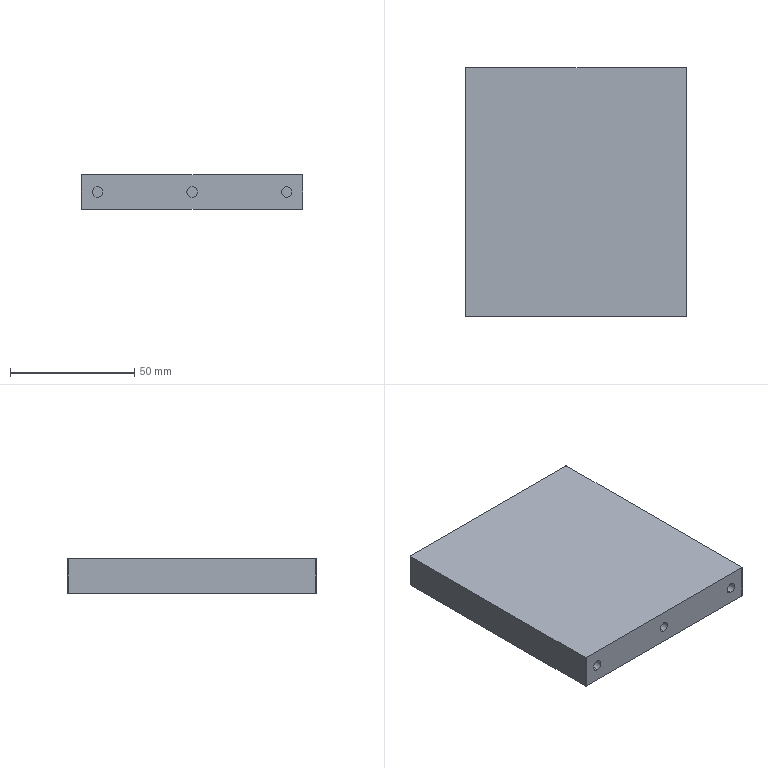CAM job | Mastercam | mm | 8 operations | part box 89 x 100 x 14
1. Facing | 20 - 63 平铣刀
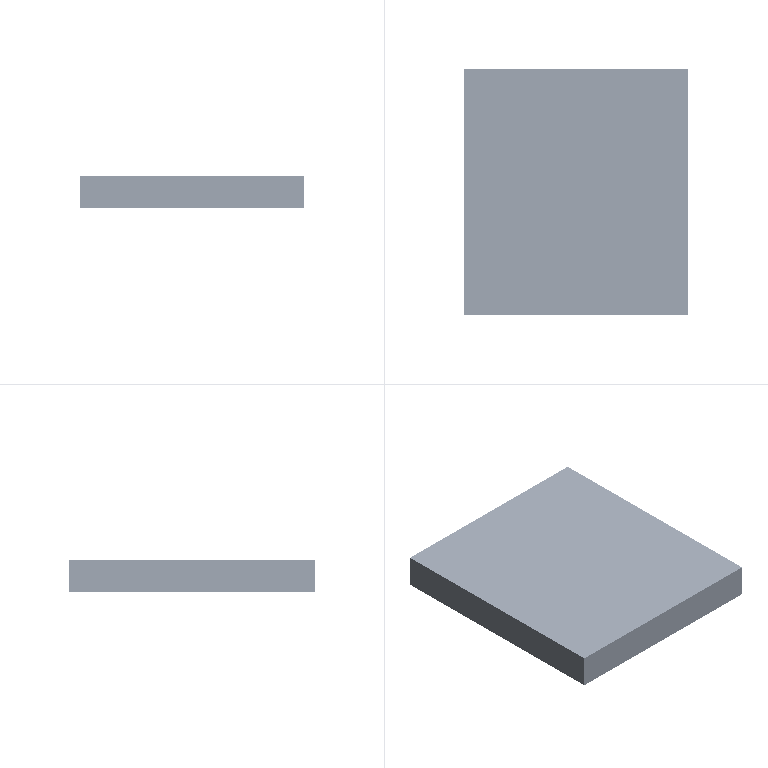2. Contour (Ramp) | 12 - 12 平铣刀
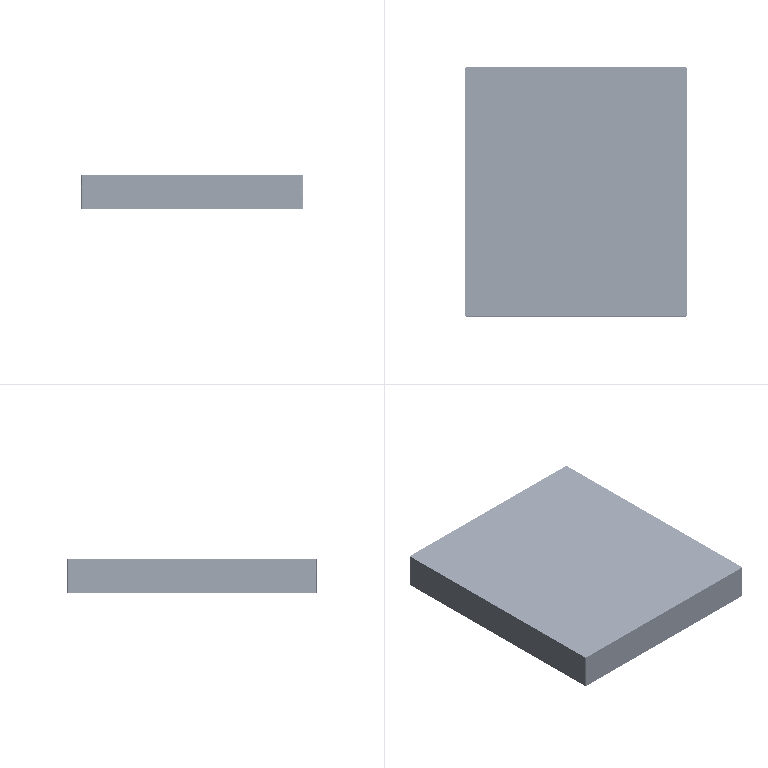3. Contour (2D) | 12 - 12 平铣刀
4. Contour (2D chamfer) | 7 - 4 倒角刀
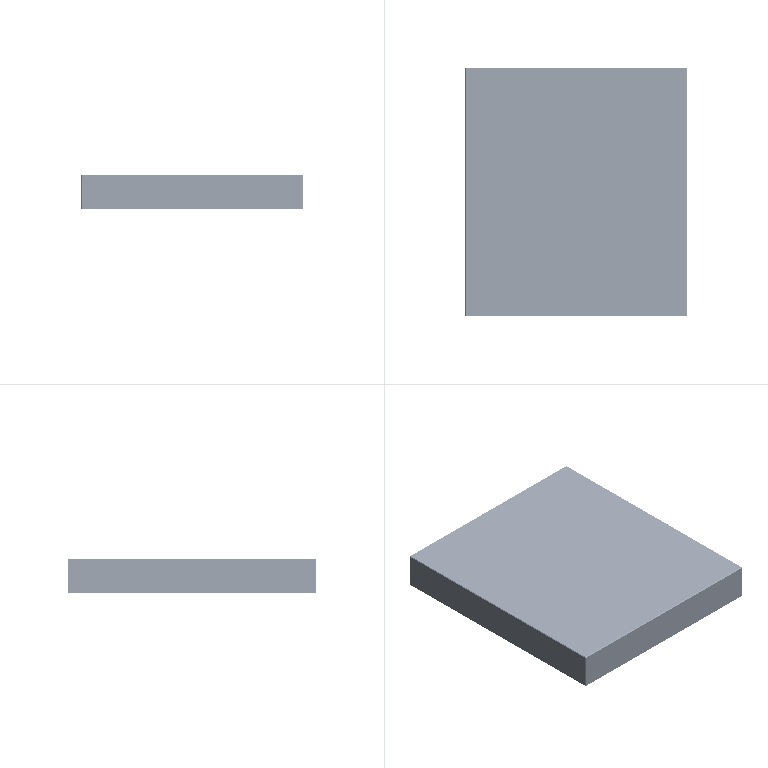5. Facing | 20 - 63 平铣刀
6. Contour (2D chamfer) | 7 - 4 倒角刀
7. Drill/Counterbore | 7 - 4 倒角刀
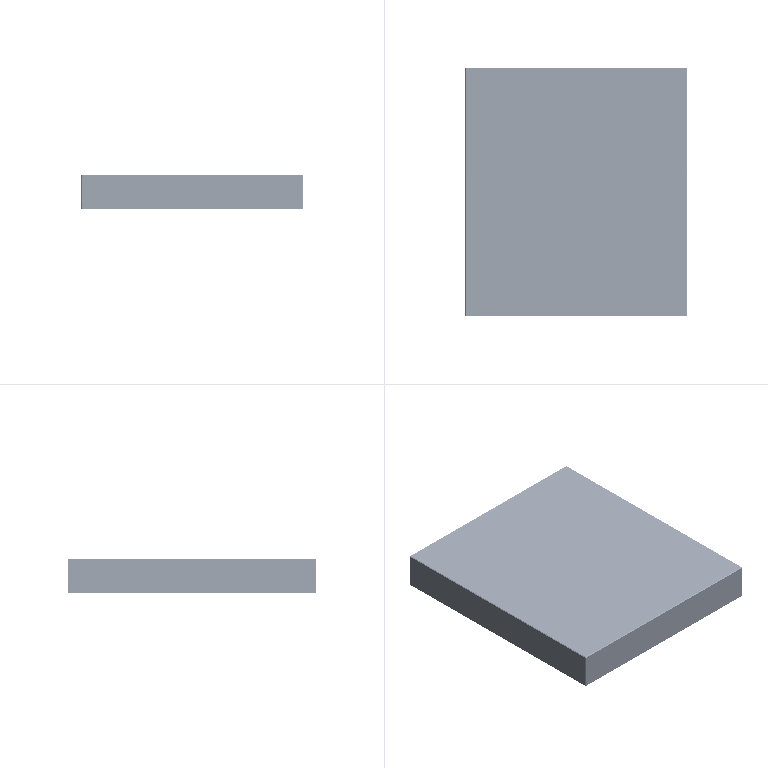8. Drill/Counterbore | 7 - 4 倒角刀